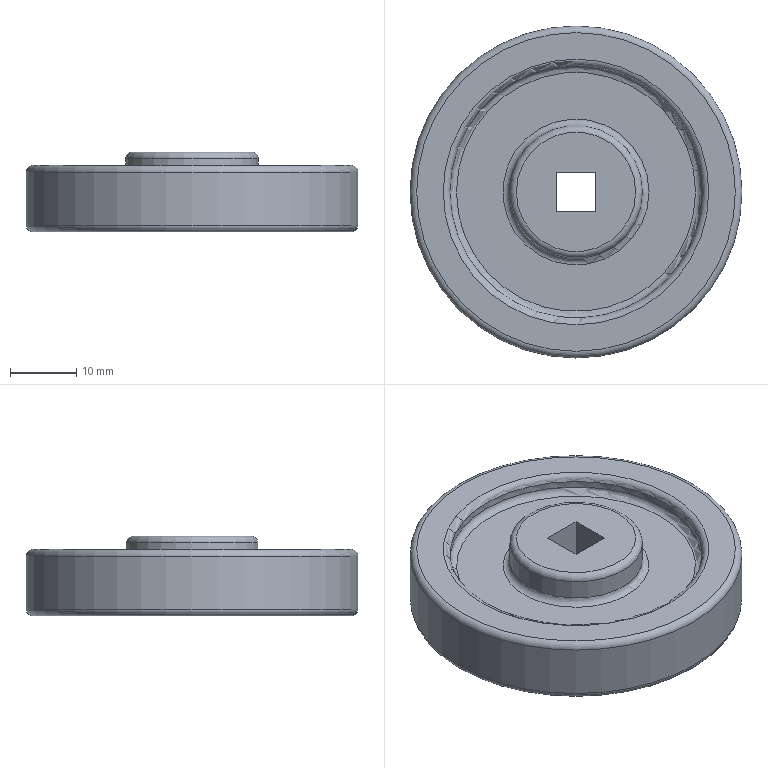Component | NX | HANDWHEEL | 1 solid | 25 faces | volume 14845 mm3 | plane 10 | torus 10 | cylinder 5 | commonest cylinder face diameters 38 x2 20 x2 50 x1